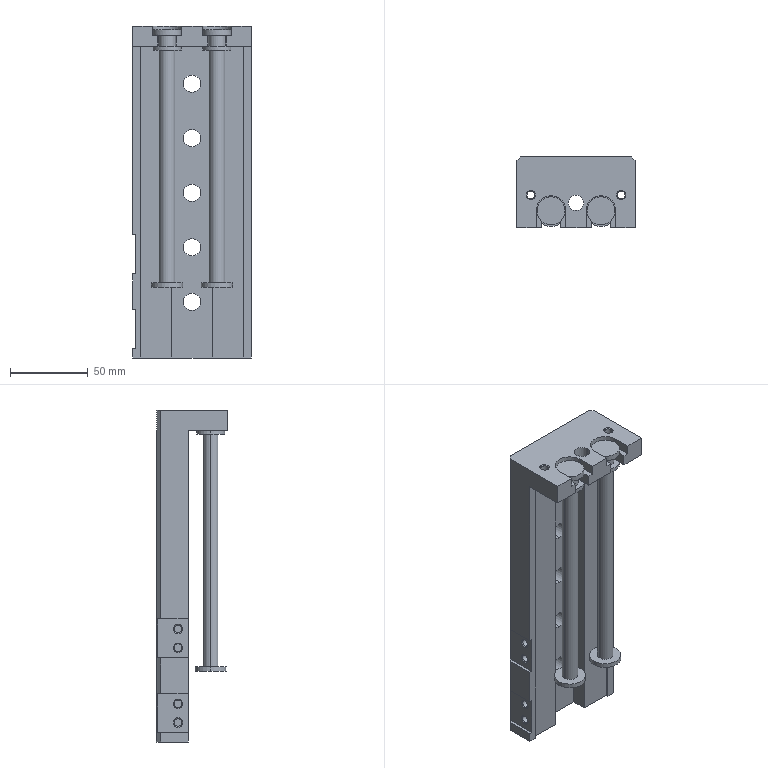Component | SolidWorks | SMC-MXS20-100AS-M9N-1_0SMC-MXS20-100AS-M9N-3-1 | 1 solid | 161 faces | box 76 x 46 x 213 mm | volume 295203 mm3 | plane 72 | cylinder 65 | cone 24 | commonest cylinder face diameters 11 x14 4.917 x12 4.134 x12 18 x8 10 x6 5 x5 20 x4 19 x2
build123d program:
from build123d import *

# Parameters (mm, degrees)
BOSS_EXTRUDE1_DEPTH  = 200
BOSS_EXTRUDE2_DEPTH  = 13
CUT_EXTRUDE1_DEPTH   = 6
CUT_EXTRUDE2_DEPTH   = 13
SKETCH7_R            = 2.5
CUT_EXTRUDE3_DEPTH   = 5.5
CUT_EXTRUDE4_DEPTH   = 5.5
LPATTERN1_COUNT      = 2
LPATTERN1_PITCH      = 46
LPATTERN1_COUNT_DIR2 = 3
LPATTERN1_PITCH_DIR2 = 70
SKETCH13_R           = 5
CUT_EXTRUDE5_DEPTH   = 13
SKETCH14_R           = 5.5
CUT_EXTRUDE6_DEPTH   = 50
SKETCH15_R           = 5.5
CUT_EXTRUDE7_DEPTH   = 50
SKETCH16_R           = 5.5
CUT_EXTRUDE8_DEPTH   = 50
SKETCH17_R           = 5.5
CUT_EXTRUDE9_DEPTH   = 50
SKETCH18_R           = 5.5
CUT_EXTRUDE10_DEPTH  = 50
SKETCH21_W           = 2
SKETCH21_H           = 25
CUT_EXTRUDE11_DEPTH  = 50
SKETCH24_W           = 2
SKETCH24_H           = 25
CUT_EXTRUDE12_DEPTH  = 50
SKETCH27_W           = 9
SKETCH27_H           = 2.5
SKETCH28_W           = 9
SKETCH28_H           = 2.5


with BuildPart() as part:
    # Sketch1 → Boss-Extrude1 (new body)
    with BuildSketch(Plane.XY.offset(201)):
        Polygon((-38, 29.5), (-33, 29.5), (-33, 31), (-13, 31), (-13, 40.5), (13, 40.5), (13, 31), (33, 31), (33, 29.5), (38, 29.5), (38, 47), (35.5, 49.5), (31, 49.5), (30.5, 50), (15.5, 50), (15, 49.5), (-15, 49.5), (-15.5, 50), (-30.5, 50), (-31, 49.5), (-35.5, 49.5), (-38, 47), align=None)
    extrude(amount=-BOSS_EXTRUDE1_DEPTH)

    # Sketch2 → Boss-Extrude2 (add)
    with BuildSketch(Plane.XY.offset(201)):
        Polygon((-38, 4), (38, 4), (38, 47), (35.5, 49.5), (-35.5, 49.5), (-38, 47), align=None)
    extrude(amount=BOSS_EXTRUDE2_DEPTH)

    # Sketch3 → Cut-Extrude1 (cut)
    with BuildSketch(Plane.XY.offset(214)):
        with BuildLine():
            Line((-25.5, 0), (25.5, 0))
            Line((25.5, 0), (25.5, 15))
            ThreePointArc((25.5, 15), (16, 24.5), (6.5, 15))
            Line((6.5, 15), (6.5, 1))
            Line((6.5, 1), (-6.5, 1))
            Line((-6.5, 1), (-6.5, 15))
            ThreePointArc((-6.5, 15), (-16, 24.5), (-25.5, 15))
            Line((-25.5, 15), (-25.5, 0))
        make_face()
    extrude(amount=-CUT_EXTRUDE1_DEPTH, mode=Mode.SUBTRACT)

    # Sketch4 → Cut-Extrude2 (cut)
    with BuildSketch(Plane.XY.offset(214)):
        with BuildLine():
            Line((-22, 15), (-22, 0))
            Line((-22, 0), (22, 0))
            Line((22, 0), (22, 15))
            ThreePointArc((22, 15), (16, 21), (10, 15))
            Line((10, 15), (10, 1))
            Line((10, 1), (-10, 1))
            Line((-10, 1), (-10, 15))
            ThreePointArc((-10, 15), (-16, 21), (-22, 15))
        make_face()
    extrude(amount=-CUT_EXTRUDE2_DEPTH, mode=Mode.SUBTRACT)

    # Sketch5 → Revolve1 (revolve)
    with BuildSketch(Plane(origin=(0, 15, 0), x_dir=(1, 0, 0), z_dir=(0, 1, 0)), mode=Mode.PRIVATE) as revolve1_sk:
        Polygon((-16, -211.5), (-25, -211.5), (-25, -208), (-21.5, -208), (-21.5, -201), (-16, -201), align=None)
    revolve(revolve1_sk.sketch.rotate(Axis((-16, 15, 201), (0, 0, 1)), 180), axis=Axis((-16, 15, 201), (0, 0, 1)))

    # Sketch6 → Revolve2 (revolve)
    with BuildSketch(Plane(origin=(0, 15, 0), x_dir=(1, 0, 0), z_dir=(0, 1, 0)), mode=Mode.PRIVATE) as revolve2_sk:
        Polygon((16, -211.5), (7, -211.5), (7, -208), (10.5, -208), (10.5, -201), (16, -201), align=None)
    revolve(revolve2_sk.sketch.rotate(Axis((16, 15, 201), (0, 0, 1)), 180), axis=Axis((16, 15, 201), (0, 0, 1)))

    # Sketch7 → Cut-Extrude3 (cut)
    with BuildSketch(Plane(origin=(0, 50, 0), x_dir=(1, 0, 0), z_dir=(0, 1, 0))):
        with Locations(Location((0, -187, 0), (0, 0, 270))):
            Circle(SKETCH7_R)
    extrude(amount=-CUT_EXTRUDE3_DEPTH, mode=Mode.SUBTRACT)

    # Sketch8 → Cut-Extrude4 (cut)
    with BuildSketch(Plane(origin=(0, 50, 0), x_dir=(1, 0, 0), z_dir=(0, 1, 0))):
        with BuildLine():
            Line((-2.5, -116.5), (-2.5, -117.5))
            ThreePointArc((-2.5, -117.5), (0, -120), (2.5, -117.5))
            Line((2.5, -117.5), (2.5, -116.5))
            ThreePointArc((2.5, -116.5), (0, -114), (-2.5, -116.5))
        make_face()
    extrude(amount=-CUT_EXTRUDE4_DEPTH, mode=Mode.SUBTRACT)

    # Sketch9 → Cut-Revolve1 (revolve, cut)
    with BuildSketch(Plane.XY.offset(187), mode=Mode.PRIVATE) as cut_revolve1_sk:
        Polygon((-23, 40), (-25.067, 40), (-25.067, 49.567), (-25.5, 50), (-23, 50), align=None)
    cut_revolve1 = revolve(cut_revolve1_sk.sketch.rotate(Axis((-23, 50, 187), (0, -1, 0)), 90), axis=Axis((-23, 50, 187), (0, -1, 0)), mode=Mode.SUBTRACT)

    # LPattern1: Cut-Revolve1 2 × 3
    with Locations(*[(i * LPATTERN1_PITCH, 0, -j * LPATTERN1_PITCH_DIR2) for i in range(LPATTERN1_COUNT) for j in range(LPATTERN1_COUNT_DIR2) if (i, j) != (0, 0)]):
        add(cut_revolve1, mode=Mode.SUBTRACT)

    # Sketch11 → Cut-Revolve2 (revolve, cut)
    with BuildSketch(Plane(origin=(0, 25, 0), x_dir=(1, 0, 0), z_dir=(0, 1, 0)), mode=Mode.PRIVATE) as cut_revolve2_sk:
        Polygon((-29, -214), (-32, -214), (-31.459, -213.458), (-31.459, -201), (-29, -201), align=None)
    revolve(cut_revolve2_sk.sketch.rotate(Axis((-29, 25, 201), (0, 0, 1)), 180), axis=Axis((-29, 25, 201), (0, 0, 1)), mode=Mode.SUBTRACT)

    # Sketch12 → Cut-Revolve3 (revolve, cut)
    with BuildSketch(Plane(origin=(0, 25, 0), x_dir=(1, 0, 0), z_dir=(0, 1, 0)), mode=Mode.PRIVATE) as cut_revolve3_sk:
        Polygon((29, -214), (26, -214), (26.541, -213.458), (26.541, -201), (29, -201), align=None)
    revolve(cut_revolve3_sk.sketch.rotate(Axis((29, 25, 201), (0, 0, 1)), 180), axis=Axis((29, 25, 201), (0, 0, 1)), mode=Mode.SUBTRACT)

    # Sketch13 → Cut-Extrude5 (cut)
    with BuildSketch(Plane.XY.offset(214)):
        with Locations((0, 20)):
            Circle(SKETCH13_R)
    extrude(amount=-CUT_EXTRUDE5_DEPTH, mode=Mode.SUBTRACT)

    # Sketch14 → Cut-Extrude6 (cut)
    with BuildSketch(Plane(origin=(0, 0, 0), x_dir=(1, 0, 0), z_dir=(0, 1, 0))):
        with Locations(Location((0, -177, 0), (0, 0, 90))):
            Circle(SKETCH14_R)
    extrude(amount=CUT_EXTRUDE6_DEPTH, mode=Mode.SUBTRACT)

    # Sketch15 → Cut-Extrude7 (cut)
    with BuildSketch(Plane(origin=(0, 0, 0), x_dir=(1, 0, 0), z_dir=(0, 1, 0))):
        with Locations(Location((0, -37, 0), (0, 0, 90))):
            Circle(SKETCH15_R)
    extrude(amount=CUT_EXTRUDE7_DEPTH, mode=Mode.SUBTRACT)

    # Sketch16 → Cut-Extrude8 (cut)
    with BuildSketch(Plane(origin=(0, 0, 0), x_dir=(1, 0, 0), z_dir=(0, 1, 0))):
        with Locations(Location((0, -72, 0), (0, 0, 90))):
            Circle(SKETCH16_R)
    extrude(amount=CUT_EXTRUDE8_DEPTH, mode=Mode.SUBTRACT)

    # Sketch17 → Cut-Extrude9 (cut)
    with BuildSketch(Plane(origin=(0, 0, 0), x_dir=(1, 0, 0), z_dir=(0, 1, 0))):
        with Locations(Location((0, -107, 0), (0, 0, 90))):
            Circle(SKETCH17_R)
    extrude(amount=CUT_EXTRUDE9_DEPTH, mode=Mode.SUBTRACT)

    # Sketch18 → Cut-Extrude10 (cut)
    with BuildSketch(Plane(origin=(0, 0, 0), x_dir=(1, 0, 0), z_dir=(0, 1, 0))):
        with Locations(Location((0, -142, 0), (0, 0, 90))):
            Circle(SKETCH18_R)
    extrude(amount=CUT_EXTRUDE10_DEPTH, mode=Mode.SUBTRACT)

    # Sketch19 → Revolve3 (revolve)
    with BuildSketch(Plane(origin=(0, 15, 0), x_dir=(1, 0, 0), z_dir=(0, 1, 0)), mode=Mode.PRIVATE) as revolve3_sk:
        Polygon((-16, -201), (-21, -201), (-21, -49.25), (-26, -49.25), (-26, -46.25), (-16, -46.25), align=None)
    revolve(revolve3_sk.sketch.rotate(Axis((-16, 15, 46.25), (0, 0, 1)), 180), axis=Axis((-16, 15, 46.25), (0, 0, 1)))

    # Sketch20 → Revolve4 (revolve)
    with BuildSketch(Plane(origin=(0, 15, 0), x_dir=(1, 0, 0), z_dir=(0, 1, 0)), mode=Mode.PRIVATE) as revolve4_sk:
        Polygon((16, -201), (11, -201), (11, -49.25), (6, -49.25), (6, -46.25), (16, -46.25), align=None)
    revolve(revolve4_sk.sketch.rotate(Axis((16, 15, 46.25), (0, 0, 1)), 180), axis=Axis((16, 15, 46.25), (0, 0, 1)))

    # Sketch21 → Cut-Extrude11 (cut)
    with BuildSketch(Plane(origin=(0, 0, 0), x_dir=(1, 0, 0), z_dir=(0, 1, 0))):
        with Locations((-37, -67.5)):
            Rectangle(SKETCH21_W, SKETCH21_H)
    extrude(amount=CUT_EXTRUDE11_DEPTH, mode=Mode.SUBTRACT)

    # Sketch22 → Cut-Revolve4 (revolve, cut)
    with BuildSketch(Plane.XY.offset(73.5), mode=Mode.PRIVATE) as cut_revolve4_sk:
        Polygon((-36, 36), (-36, 39), (-35.459, 38.459), (-29.5, 38.459), (-29.5, 36), align=None)
    revolve(cut_revolve4_sk.sketch.rotate(Axis((-29.5, 36, 73.5), (-1, 0, 0)), 270), axis=Axis((-29.5, 36, 73.5), (-1, 0, 0)), mode=Mode.SUBTRACT)

    # Sketch23 → Cut-Revolve5 (revolve, cut)
    with BuildSketch(Plane.XY.offset(61.5), mode=Mode.PRIVATE) as cut_revolve5_sk:
        Polygon((-36, 36), (-36, 39), (-35.459, 38.459), (-29.5, 38.459), (-29.5, 36), align=None)
    revolve(cut_revolve5_sk.sketch.rotate(Axis((-29.5, 36, 61.5), (-1, 0, 0)), 270), axis=Axis((-29.5, 36, 61.5), (-1, 0, 0)), mode=Mode.SUBTRACT)

    # Sketch24 → Cut-Extrude12 (cut)
    with BuildSketch(Plane(origin=(0, 0, 0), x_dir=(1, 0, 0), z_dir=(0, 1, 0))):
        with Locations((-37, -19.5)):
            Rectangle(SKETCH24_W, SKETCH24_H)
    extrude(amount=CUT_EXTRUDE12_DEPTH, mode=Mode.SUBTRACT)

    # Sketch25 → Cut-Revolve6 (revolve, cut)
    with BuildSketch(Plane.XY.offset(25.5), mode=Mode.PRIVATE) as cut_revolve6_sk:
        Polygon((-36, 36), (-36, 39), (-35.459, 38.459), (-29.5, 38.459), (-29.5, 36), align=None)
    revolve(cut_revolve6_sk.sketch.rotate(Axis((-29.5, 36, 25.5), (-1, 0, 0)), 270), axis=Axis((-29.5, 36, 25.5), (-1, 0, 0)), mode=Mode.SUBTRACT)

    # Sketch26 → Cut-Revolve7 (revolve, cut)
    with BuildSketch(Plane.XY.offset(13.5), mode=Mode.PRIVATE) as cut_revolve7_sk:
        Polygon((-36, 36), (-36, 39), (-35.459, 38.459), (-29.5, 38.459), (-29.5, 36), align=None)
    revolve(cut_revolve7_sk.sketch.rotate(Axis((-29.5, 36, 13.5), (-1, 0, 0)), 270), axis=Axis((-29.5, 36, 13.5), (-1, 0, 0)), mode=Mode.SUBTRACT)

    # Sketch27 → Revolve5 (revolve)
    with BuildSketch(Plane(origin=(0, 15, 0), x_dir=(1, 0, 0), z_dir=(0, 1, 0)), mode=Mode.PRIVATE) as revolve5_sk:
        with Locations((-20.5, -199.75)):
            Rectangle(SKETCH27_W, SKETCH27_H)
    revolve(revolve5_sk.sketch.rotate(Axis((-16, 15, 198.5), (0, 0, 1)), 180), axis=Axis((-16, 15, 198.5), (0, 0, 1)))

    # Sketch28 → Revolve6 (revolve)
    with BuildSketch(Plane(origin=(0, 15, 0), x_dir=(1, 0, 0), z_dir=(0, 1, 0)), mode=Mode.PRIVATE) as revolve6_sk:
        with Locations((11.5, -199.75)):
            Rectangle(SKETCH28_W, SKETCH28_H)
    revolve(revolve6_sk.sketch.rotate(Axis((16, 15, 198.5), (0, 0, 1)), 180), axis=Axis((16, 15, 198.5), (0, 0, 1)))


solid = part.part

# Placed as in the assembly
solid = solid.moved(Location((-235.009, 50.721, 15.089), (0, 0, 0)))